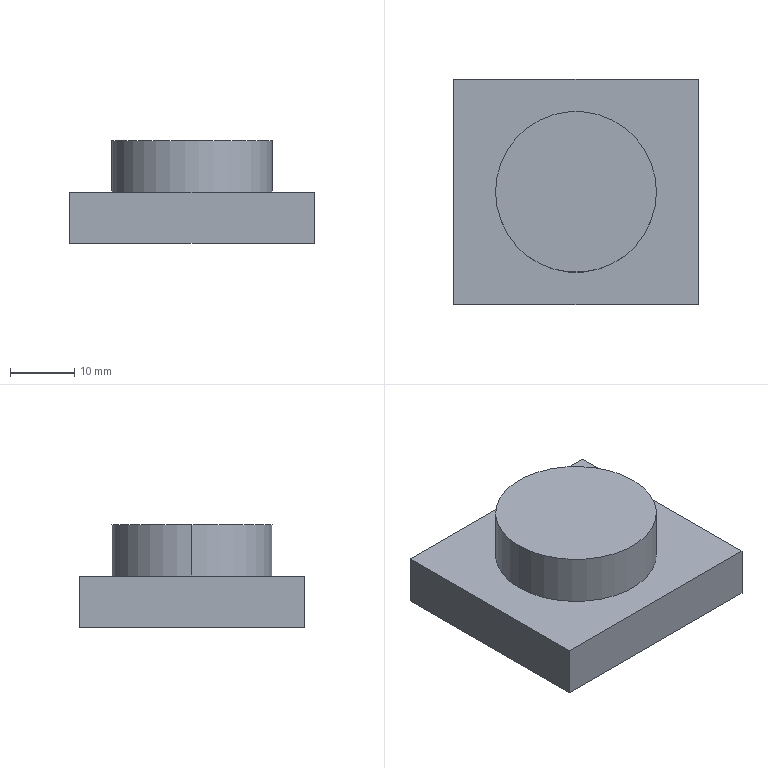Component | SolidWorks | MotorCover-1 | 1 solid | 9 faces | box 38 x 35 x 16 mm | volume 14567 mm3 | plane 7 | cylinder 2 | commonest cylinder face diameters 25 x2
build123d program:
from build123d import *

# Parameters (mm, degrees)
SKETCH1_R           = 12.5
BOSS_EXTRUDE1_DEPTH = 8
SKETCH2_W           = 38
SKETCH2_H           = 35
BOSS_EXTRUDE2_DEPTH = 8


with BuildPart() as part:
    # Sketch1 → Boss-Extrude1 (new body)
    with BuildSketch(Plane.XY):
        Circle(SKETCH1_R)
    extrude(amount=-BOSS_EXTRUDE1_DEPTH)

    # Sketch2 → Boss-Extrude2 (add)
    with BuildSketch(Plane.XY):
        Rectangle(SKETCH2_W, SKETCH2_H)
    extrude(amount=BOSS_EXTRUDE2_DEPTH)


solid = part.part

# Placed as in the assembly
solid = solid.moved(Location((-24.375, -67.172, -107.818), (180, 0, 0)))
STEP:
#1=COLOUR_RGB('',0.7922,0.8196,0.9333);
#2=FILL_AREA_STYLE_COLOUR('',#1);
#3=FILL_AREA_STYLE('',(#2));
#4=SURFACE_STYLE_FILL_AREA(#3);
#5=SURFACE_SIDE_STYLE('',(#4));
#6=SURFACE_STYLE_USAGE(.BOTH.,#5);
#7=PRESENTATION_STYLE_ASSIGNMENT((#6));
#8=CARTESIAN_POINT('',(-1.452,-2.645,-3.93));
#9=VERTEX_POINT('',#8);
#10=CARTESIAN_POINT('',(-0.4675,-2.645,-3.93));
#11=VERTEX_POINT('',#10);
#12=CARTESIAN_POINT('',(-0.9597,-2.645,-3.93));
#13=DIRECTION('',(-0.,0.,-1.));
#14=DIRECTION('',(-1.,0.,0.));
#15=AXIS2_PLACEMENT_3D('',#12,#13,#14);
#16=CIRCLE('',#15,0.4921);
#17=EDGE_CURVE('',#9,#11,#16,.T.);
#18=ORIENTED_EDGE('',*,*,#17,.T.);
#19=CARTESIAN_POINT('',(-0.4675,-2.645,-4.245));
#20=VERTEX_POINT('',#19);
#21=CARTESIAN_POINT('',(-0.4675,-2.645,-3.93));
#22=DIRECTION('',(-0.,0.,-1.));
#23=VECTOR('',#22,39.37);
#24=LINE('',#21,#23);
#25=EDGE_CURVE('',#11,#20,#24,.T.);
#26=ORIENTED_EDGE('',*,*,#25,.T.);
#27=CARTESIAN_POINT('',(-1.452,-2.645,-4.245));
#28=VERTEX_POINT('',#27);
#29=CARTESIAN_POINT('',(-0.9597,-2.645,-4.245));
#30=DIRECTION('',(-0.,0.,-1.));
#31=DIRECTION('',(-1.,0.,0.));
#32=AXIS2_PLACEMENT_3D('',#29,#30,#31);
#33=CIRCLE('',#32,0.4921);
#34=EDGE_CURVE('',#28,#20,#33,.T.);
#35=ORIENTED_EDGE('',*,*,#34,.F.);
#36=CARTESIAN_POINT('',(-1.452,-2.645,-3.93));
#37=DIRECTION('',(-0.,0.,-1.));
#38=VECTOR('',#37,39.37);
#39=LINE('',#36,#38);
#40=EDGE_CURVE('',#9,#28,#39,.T.);
#41=ORIENTED_EDGE('',*,*,#40,.F.);
#42=EDGE_LOOP('',(#18,#26,#35,#41));
#43=FACE_OUTER_BOUND('',#42,.T.);
#44=CARTESIAN_POINT('',(-0.9597,-2.645,-3.93));
#45=DIRECTION('',(-0.,0.,-1.));
#46=DIRECTION('',(-1.,0.,0.));
#47=AXIS2_PLACEMENT_3D('',#44,#45,#46);
#48=CYLINDRICAL_SURFACE('',#47,0.4921);
#49=ADVANCED_FACE('',(#43),#48,.T.);
#50=ORIENTED_EDGE('',*,*,#25,.F.);
#51=CARTESIAN_POINT('',(-0.9597,-2.645,-3.93));
#52=DIRECTION('',(-0.,0.,-1.));
#53=DIRECTION('',(-1.,0.,0.));
#54=AXIS2_PLACEMENT_3D('',#51,#52,#53);
#55=CIRCLE('',#54,0.4921);
#56=EDGE_CURVE('',#11,#9,#55,.T.);
#57=ORIENTED_EDGE('',*,*,#56,.T.);
#58=ORIENTED_EDGE('',*,*,#40,.T.);
#59=CARTESIAN_POINT('',(-0.9597,-2.645,-4.245));
#60=DIRECTION('',(-0.,0.,-1.));
#61=DIRECTION('',(-1.,0.,0.));
#62=AXIS2_PLACEMENT_3D('',#59,#60,#61);
#63=CIRCLE('',#62,0.4921);
#64=EDGE_CURVE('',#20,#28,#63,.T.);
#65=ORIENTED_EDGE('',*,*,#64,.F.);
#66=EDGE_LOOP('',(#50,#57,#58,#65));
#67=FACE_OUTER_BOUND('',#66,.T.);
#68=CARTESIAN_POINT('',(-0.9597,-2.645,-3.93));
#69=DIRECTION('',(-0.,0.,-1.));
#70=DIRECTION('',(-1.,0.,0.));
#71=AXIS2_PLACEMENT_3D('',#68,#69,#70);
#72=CYLINDRICAL_SURFACE('',#71,0.4921);
#73=ADVANCED_FACE('',(#67),#72,.T.);
#74=ORIENTED_EDGE('',*,*,#17,.F.);
#75=ORIENTED_EDGE('',*,*,#56,.F.);
#76=EDGE_LOOP('',(#74,#75));
#77=FACE_OUTER_BOUND('',#76,.T.);
#78=CARTESIAN_POINT('',(-0.9597,-2.645,-3.93));
#79=DIRECTION('',(-0.,0.,-1.));
#80=DIRECTION('',(-1.,0.,0.));
#81=AXIS2_PLACEMENT_3D('',#78,#79,#80);
#82=PLANE('',#81);
#83=ADVANCED_FACE('',(#77),#82,.F.);
#84=CARTESIAN_POINT('',(-0.2116,-1.956,-4.245));
#85=VERTEX_POINT('',#84);
#86=CARTESIAN_POINT('',(-0.2116,-3.334,-4.245));
#87=VERTEX_POINT('',#86);
#88=CARTESIAN_POINT('',(-0.2116,-3.334,-4.245));
#89=DIRECTION('',(0.,-1.,0.));
#90=VECTOR('',#89,39.37);
#91=LINE('',#88,#90);
#92=EDGE_CURVE('',#85,#87,#91,.T.);
#93=ORIENTED_EDGE('',*,*,#92,.T.);
#94=CARTESIAN_POINT('',(-0.2116,-3.334,-4.56));
#95=VERTEX_POINT('',#94);
#96=CARTESIAN_POINT('',(-0.2116,-3.334,-4.56));
#97=DIRECTION('',(0.,0.,1.));
#98=VECTOR('',#97,39.37);
#99=LINE('',#96,#98);
#100=EDGE_CURVE('',#95,#87,#99,.T.);
#101=ORIENTED_EDGE('',*,*,#100,.F.);
#102=CARTESIAN_POINT('',(-0.2116,-1.956,-4.56));
#103=VERTEX_POINT('',#102);
#104=CARTESIAN_POINT('',(-0.2116,-3.334,-4.56));
#105=DIRECTION('',(0.,-1.,0.));
#106=VECTOR('',#105,39.37);
#107=LINE('',#104,#106);
#108=EDGE_CURVE('',#103,#95,#107,.T.);
#109=ORIENTED_EDGE('',*,*,#108,.F.);
#110=CARTESIAN_POINT('',(-0.2116,-1.956,-4.56));
#111=DIRECTION('',(0.,0.,1.));
#112=VECTOR('',#111,39.37);
#113=LINE('',#110,#112);
#114=EDGE_CURVE('',#103,#85,#113,.T.);
#115=ORIENTED_EDGE('',*,*,#114,.T.);
#116=EDGE_LOOP('',(#93,#101,#109,#115));
#117=FACE_OUTER_BOUND('',#116,.T.);
#118=CARTESIAN_POINT('',(-0.2116,-3.334,-4.56));
#119=DIRECTION('',(-1.,0.,0.));
#120=DIRECTION('',(0.,0.,1.));
#121=AXIS2_PLACEMENT_3D('',#118,#119,#120);
#122=PLANE('',#121);
#123=ADVANCED_FACE('',(#117),#122,.F.);
#124=CARTESIAN_POINT('',(-1.708,-3.334,-4.245));
#125=VERTEX_POINT('',#124);
#126=CARTESIAN_POINT('',(-1.708,-3.334,-4.245));
#127=DIRECTION('',(-1.,0.,0.));
#128=VECTOR('',#127,39.37);
#129=LINE('',#126,#128);
#130=EDGE_CURVE('',#87,#125,#129,.T.);
#131=ORIENTED_EDGE('',*,*,#130,.T.);
#132=CARTESIAN_POINT('',(-1.708,-3.334,-4.56));
#133=VERTEX_POINT('',#132);
#134=CARTESIAN_POINT('',(-1.708,-3.334,-4.56));
#135=DIRECTION('',(0.,0.,1.));
#136=VECTOR('',#135,39.37);
#137=LINE('',#134,#136);
#138=EDGE_CURVE('',#133,#125,#137,.T.);
#139=ORIENTED_EDGE('',*,*,#138,.F.);
#140=CARTESIAN_POINT('',(-1.708,-3.334,-4.56));
#141=DIRECTION('',(-1.,0.,0.));
#142=VECTOR('',#141,39.37);
#143=LINE('',#140,#142);
#144=EDGE_CURVE('',#95,#133,#143,.T.);
#145=ORIENTED_EDGE('',*,*,#144,.F.);
#146=ORIENTED_EDGE('',*,*,#100,.T.);
#147=EDGE_LOOP('',(#131,#139,#145,#146));
#148=FACE_OUTER_BOUND('',#147,.T.);
#149=CARTESIAN_POINT('',(-1.708,-3.334,-4.56));
#150=DIRECTION('',(0.,1.,-0.));
#151=DIRECTION('',(1.,-0.,-0.));
#152=AXIS2_PLACEMENT_3D('',#149,#150,#151);
#153=PLANE('',#152);
#154=ADVANCED_FACE('',(#148),#153,.F.);
#155=CARTESIAN_POINT('',(-1.708,-1.956,-4.245));
#156=VERTEX_POINT('',#155);
#157=CARTESIAN_POINT('',(-1.708,-3.334,-4.245));
#158=DIRECTION('',(0.,1.,0.));
#159=VECTOR('',#158,39.37);
#160=LINE('',#157,#159);
#161=EDGE_CURVE('',#125,#156,#160,.T.);
#162=ORIENTED_EDGE('',*,*,#161,.T.);
#163=CARTESIAN_POINT('',(-1.708,-1.956,-4.56));
#164=VERTEX_POINT('',#163);
#165=CARTESIAN_POINT('',(-1.708,-1.956,-4.56));
#166=DIRECTION('',(0.,0.,1.));
#167=VECTOR('',#166,39.37);
#168=LINE('',#165,#167);
#169=EDGE_CURVE('',#164,#156,#168,.T.);
#170=ORIENTED_EDGE('',*,*,#169,.F.);
#171=CARTESIAN_POINT('',(-1.708,-3.334,-4.56));
#172=DIRECTION('',(0.,1.,0.));
#173=VECTOR('',#172,39.37);
#174=LINE('',#171,#173);
#175=EDGE_CURVE('',#133,#164,#174,.T.);
#176=ORIENTED_EDGE('',*,*,#175,.F.);
#177=ORIENTED_EDGE('',*,*,#138,.T.);
#178=EDGE_LOOP('',(#162,#170,#176,#177));
#179=FACE_OUTER_BOUND('',#178,.T.);
#180=CARTESIAN_POINT('',(-1.708,-3.334,-4.56));
#181=DIRECTION('',(1.,0.,-0.));
#182=DIRECTION('',(-0.,0.,-1.));
#183=AXIS2_PLACEMENT_3D('',#180,#181,#182);
#184=PLANE('',#183);
#185=ADVANCED_FACE('',(#179),#184,.F.);
#186=CARTESIAN_POINT('',(-1.708,-1.956,-4.245));
#187=DIRECTION('',(1.,-0.,-0.));
#188=VECTOR('',#187,39.37);
#189=LINE('',#186,#188);
#190=EDGE_CURVE('',#156,#85,#189,.T.);
#191=ORIENTED_EDGE('',*,*,#190,.T.);
#192=ORIENTED_EDGE('',*,*,#114,.F.);
#193=CARTESIAN_POINT('',(-1.708,-1.956,-4.56));
#194=DIRECTION('',(1.,-0.,-0.));
#195=VECTOR('',#194,39.37);
#196=LINE('',#193,#195);
#197=EDGE_CURVE('',#164,#103,#196,.T.);
#198=ORIENTED_EDGE('',*,*,#197,.F.);
#199=ORIENTED_EDGE('',*,*,#169,.T.);
#200=EDGE_LOOP('',(#191,#192,#198,#199));
#201=FACE_OUTER_BOUND('',#200,.T.);
#202=CARTESIAN_POINT('',(-1.708,-1.956,-4.56));
#203=DIRECTION('',(-0.,-1.,0.));
#204=DIRECTION('',(-1.,0.,0.));
#205=AXIS2_PLACEMENT_3D('',#202,#203,#204);
#206=PLANE('',#205);
#207=ADVANCED_FACE('',(#201),#206,.F.);
#208=ORIENTED_EDGE('',*,*,#108,.T.);
#209=ORIENTED_EDGE('',*,*,#144,.T.);
#210=ORIENTED_EDGE('',*,*,#175,.T.);
#211=ORIENTED_EDGE('',*,*,#197,.T.);
#212=EDGE_LOOP('',(#208,#209,#210,#211));
#213=FACE_OUTER_BOUND('',#212,.T.);
#214=CARTESIAN_POINT('',(-0.9597,-2.645,-4.56));
#215=DIRECTION('',(-0.,0.,-1.));
#216=DIRECTION('',(-1.,0.,0.));
#217=AXIS2_PLACEMENT_3D('',#214,#215,#216);
#218=PLANE('',#217);
#219=ADVANCED_FACE('',(#213),#218,.T.);
#220=ORIENTED_EDGE('',*,*,#34,.T.);
#221=ORIENTED_EDGE('',*,*,#64,.T.);
#222=EDGE_LOOP('',(#220,#221));
#223=FACE_BOUND('',#222,.T.);
#224=ORIENTED_EDGE('',*,*,#92,.F.);
#225=ORIENTED_EDGE('',*,*,#190,.F.);
#226=ORIENTED_EDGE('',*,*,#161,.F.);
#227=ORIENTED_EDGE('',*,*,#130,.F.);
#228=EDGE_LOOP('',(#224,#225,#226,#227));
#229=FACE_OUTER_BOUND('',#228,.T.);
#230=CARTESIAN_POINT('',(-0.9597,-2.645,-4.245));
#231=DIRECTION('',(-0.,0.,-1.));
#232=DIRECTION('',(-1.,0.,0.));
#233=AXIS2_PLACEMENT_3D('',#230,#231,#232);
#234=PLANE('',#233);
#235=ADVANCED_FACE('',(#223,#229),#234,.F.);
#236=CLOSED_SHELL('',(#49,#73,#83,#123,#154,#185,#207,#219,#235));
#237=MANIFOLD_SOLID_BREP('',#236);
#238=STYLED_ITEM('',(#7),#237);
#239=PRESENTATION_LAYER_ASSIGNMENT('','',(#238));
#240=(LENGTH_UNIT()NAMED_UNIT(*)SI_UNIT($,.METRE.));
#241=LENGTH_MEASURE_WITH_UNIT(LENGTH_MEASURE(0.0254),#240);
#242=DIMENSIONAL_EXPONENTS(1.,0.,0.,0.,0.,0.,0.);
#243=(CONVERSION_BASED_UNIT('',#241)LENGTH_UNIT()NAMED_UNIT(#242));
#244=UNCERTAINTY_MEASURE_WITH_UNIT(LENGTH_MEASURE(0.00001),#243,'','');
#245=(NAMED_UNIT(*)PLANE_ANGLE_UNIT()SI_UNIT($,.RADIAN.));
#246=(NAMED_UNIT(*)SI_UNIT($,.STERADIAN.)SOLID_ANGLE_UNIT());
#247=(GEOMETRIC_REPRESENTATION_CONTEXT(3)GLOBAL_UNCERTAINTY_ASSIGNED_CONTEXT((#244))GLOBAL_UNIT_ASSIGNED_CONTEXT((#243,#245,#246))REPRESENTATION_CONTEXT('',''));
#248=MECHANICAL_DESIGN_GEOMETRIC_PRESENTATION_REPRESENTATION('',(#238),#247);
#249=CARTESIAN_POINT('',(0.,0.,0.));
#250=DIRECTION('',(0.,0.,1.));
#251=DIRECTION('',(1.,0.,0.));
#252=AXIS2_PLACEMENT_3D('',#249,#250,#251);
#253=(LENGTH_UNIT()NAMED_UNIT(*)SI_UNIT($,.METRE.));
#254=LENGTH_MEASURE_WITH_UNIT(LENGTH_MEASURE(0.0254),#253);
#255=DIMENSIONAL_EXPONENTS(1.,0.,0.,0.,0.,0.,0.);
#256=(CONVERSION_BASED_UNIT('',#254)LENGTH_UNIT()NAMED_UNIT(#255));
#257=UNCERTAINTY_MEASURE_WITH_UNIT(LENGTH_MEASURE(0.00001),#256,'','');
#258=(NAMED_UNIT(*)PLANE_ANGLE_UNIT()SI_UNIT($,.RADIAN.));
#259=(NAMED_UNIT(*)SI_UNIT($,.STERADIAN.)SOLID_ANGLE_UNIT());
#260=(GEOMETRIC_REPRESENTATION_CONTEXT(3)GLOBAL_UNCERTAINTY_ASSIGNED_CONTEXT((#257))GLOBAL_UNIT_ASSIGNED_CONTEXT((#256,#258,#259))REPRESENTATION_CONTEXT('',''));
#261=ADVANCED_BREP_SHAPE_REPRESENTATION('',(#237,#252),#260);